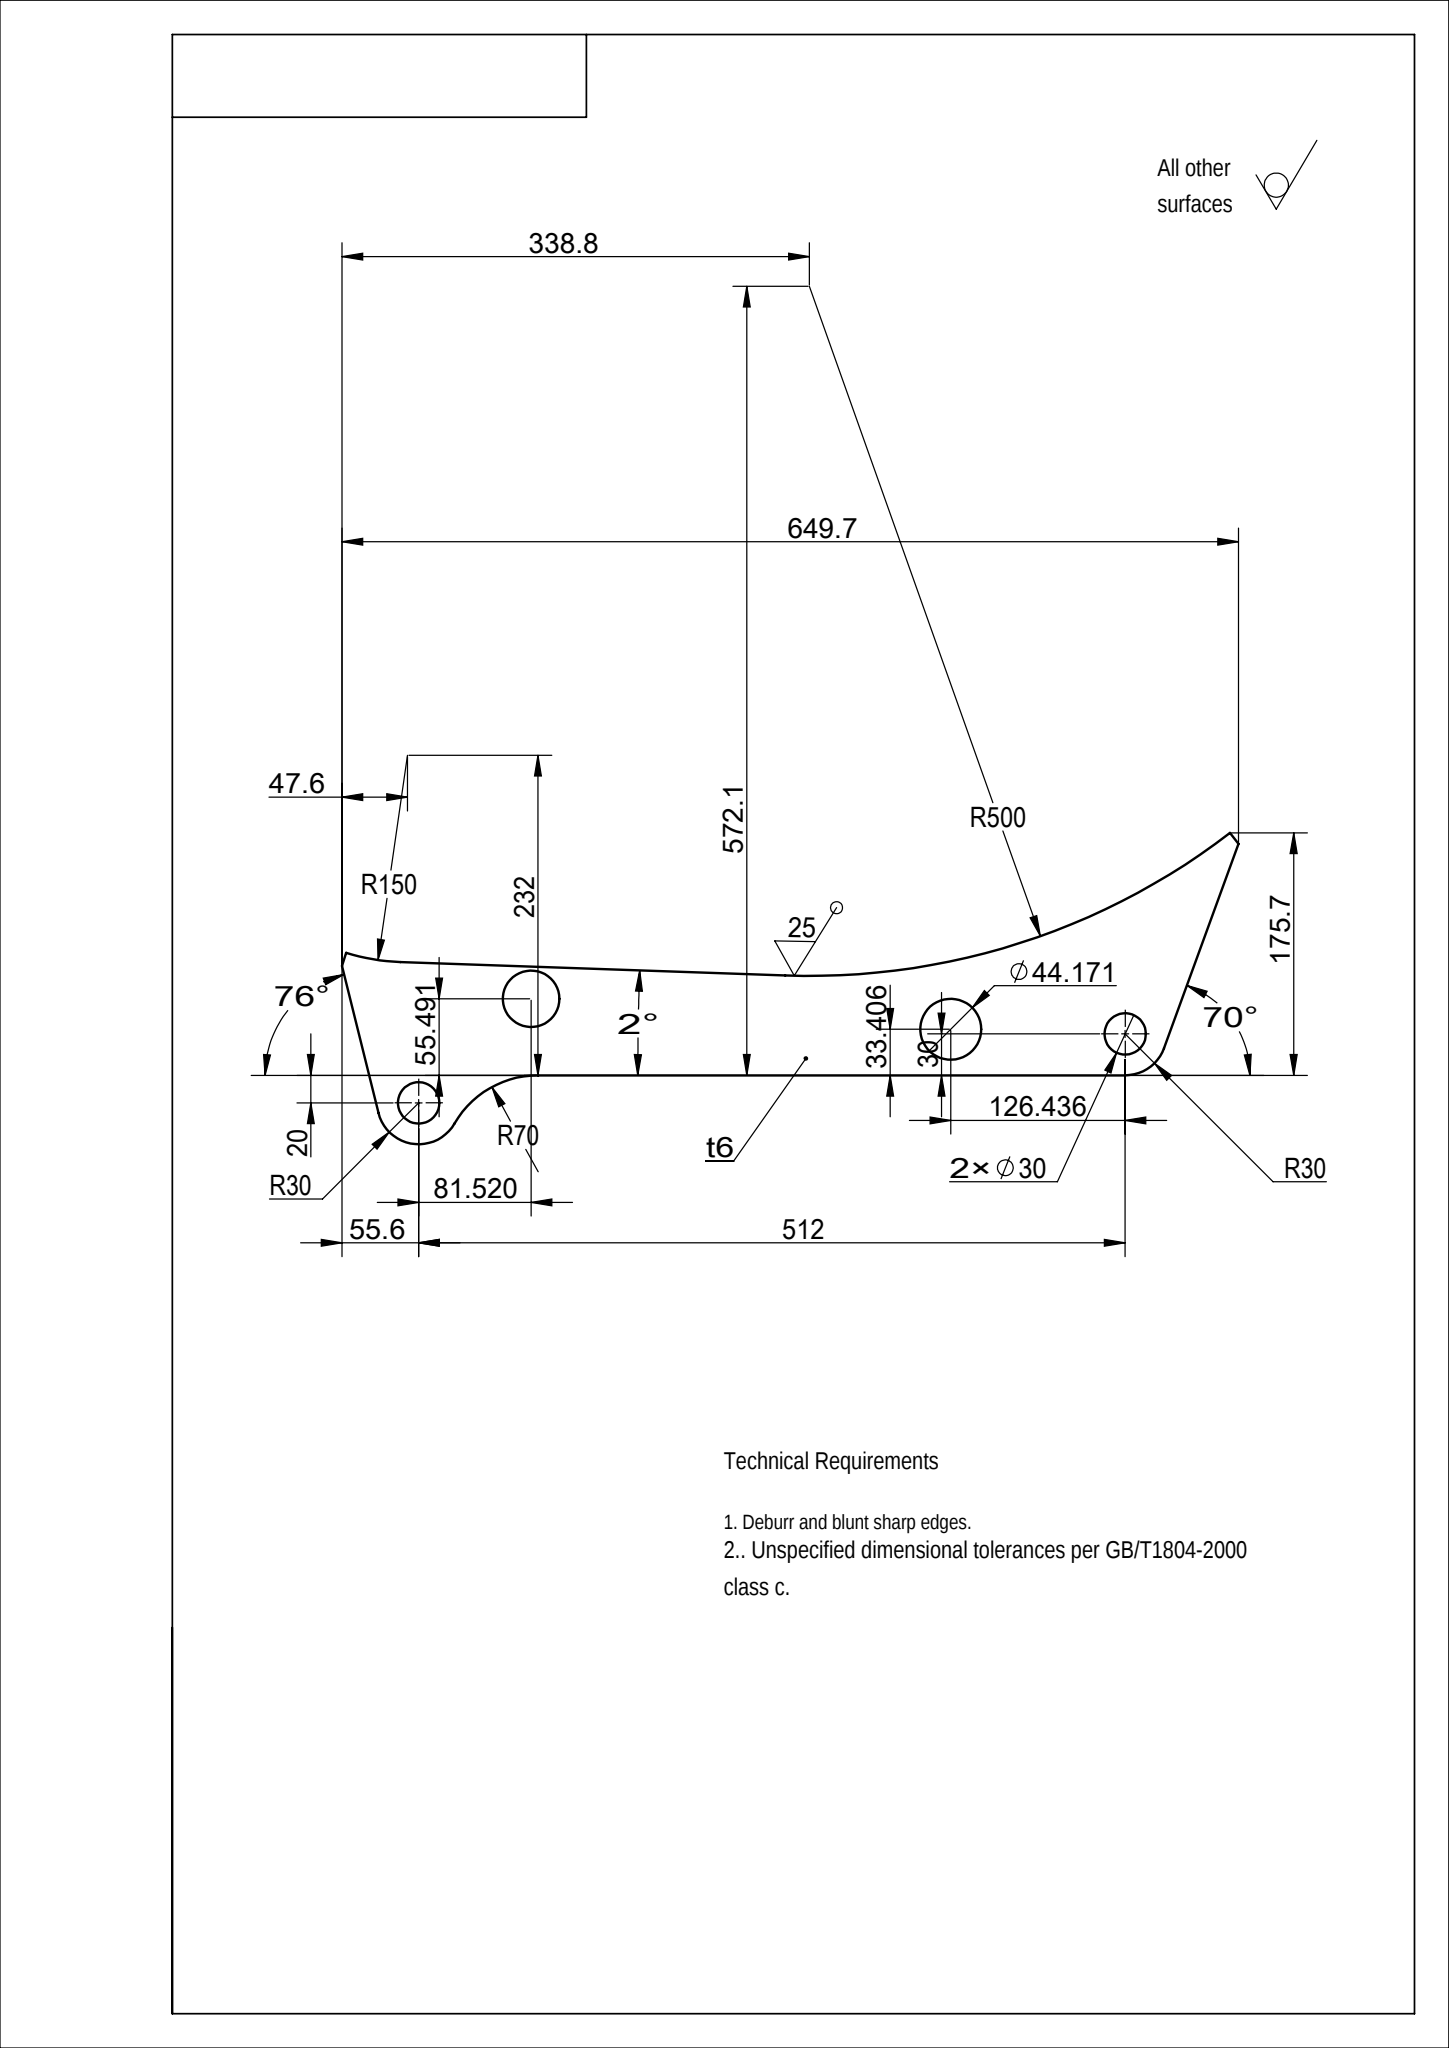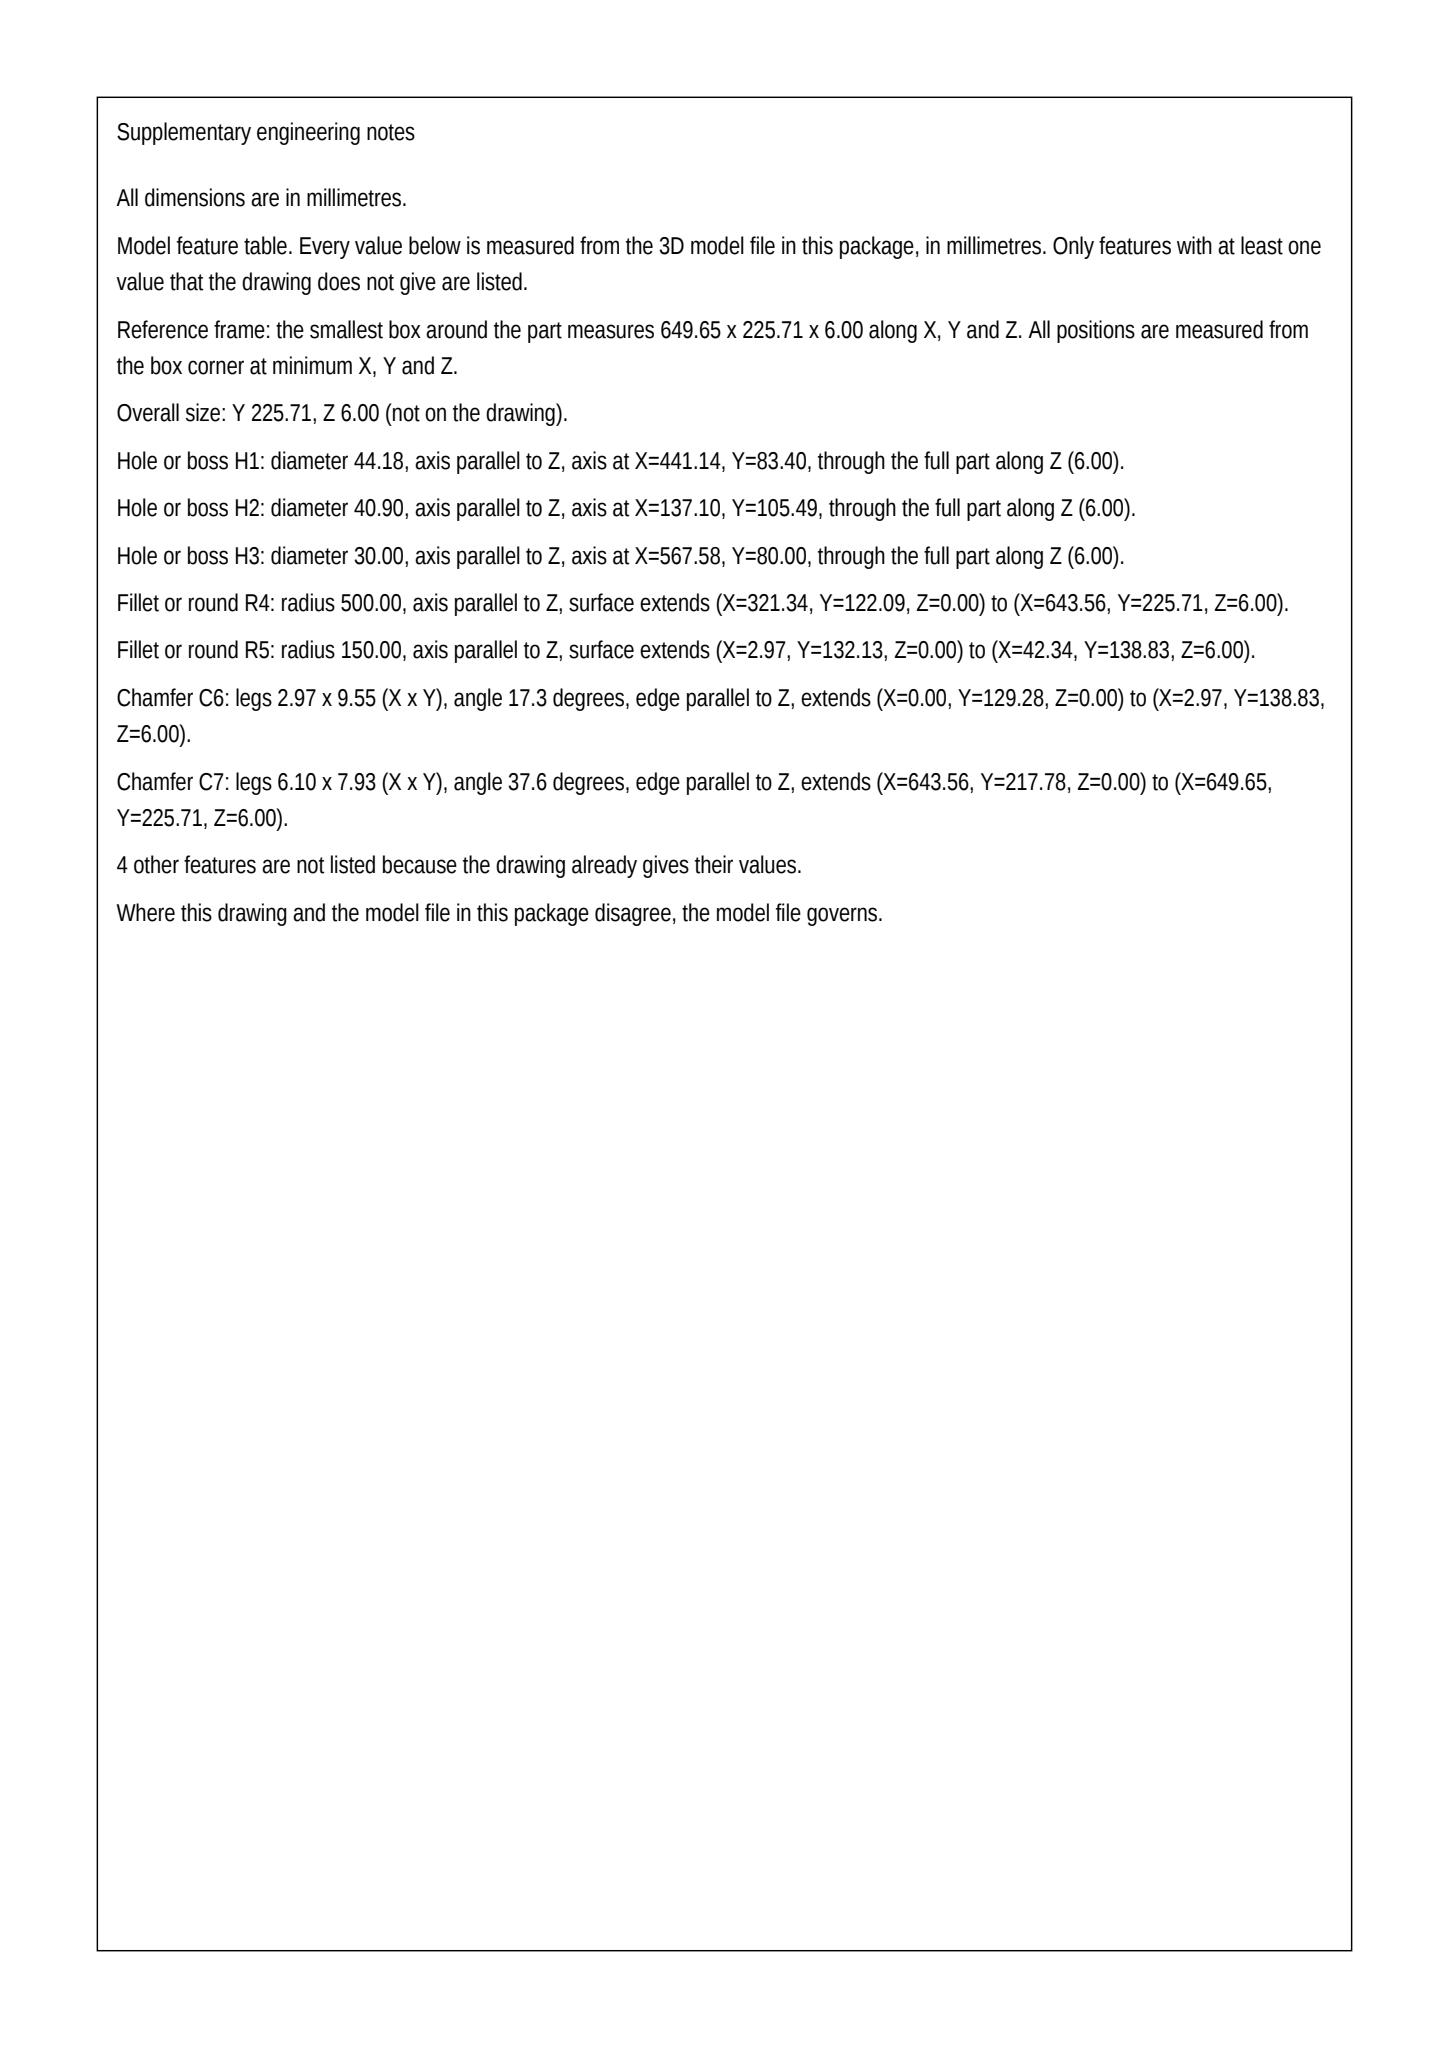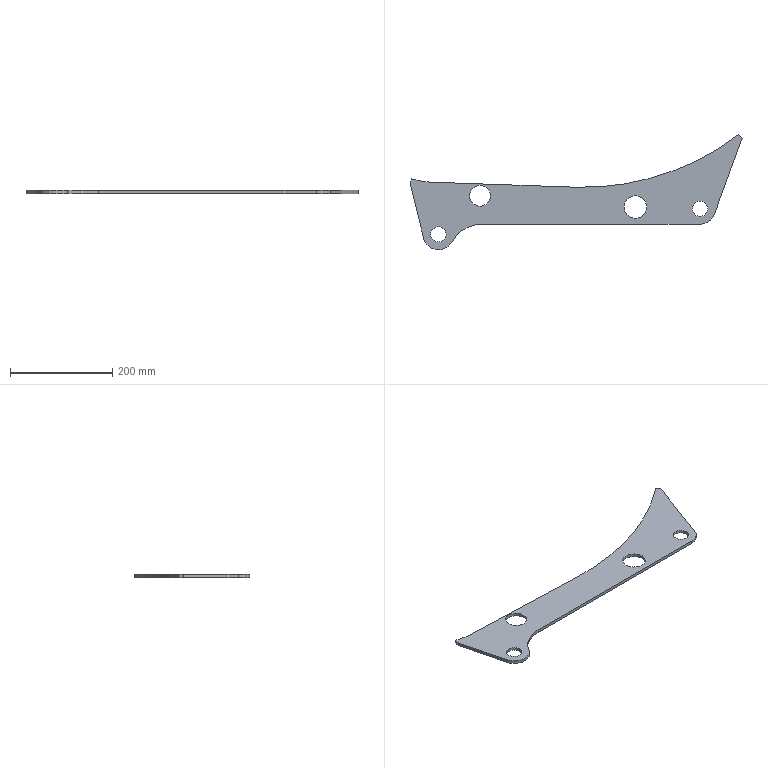Part | SolidWorks | mm | 1 solid | 21 faces | box 649.65 x 225.71 x 6 mm | volume 314367 mm3 | cylinder 13 | plane 8 | commonest cylinder face diameters 30 x4 44.171 x2 40.91 x2 60 x2 140 x1 1000 x1 300 x1
build123d program:
from build123d import *

# Parameters (mm, degrees)
BOSS_EXTRUDE1_START = 250
SKETCH1_R           = 15
BOSS_EXTRUDE1_DEPTH = 6
SKETCH3_R           = 22.086
SKETCH3_R_2         = 20.455
CUT_EXTRUDE2_DEPTH  = 80


with BuildPart() as part:
    # Sketch1 → Boss-Extrude1 (new body)
    with BuildSketch(Plane.XY.offset(BOSS_EXTRUDE1_START)):
        with BuildLine():
            Line((105.394, -627.925), (102.421, -637.473))
            Line((102.421, -637.473), (107.706, -658.746))
            Line((107.706, -658.746), (128.885, -743.987))
            ThreePointArc((128.885, -743.987), (153.813, -766.46), (183.981, -751.753))
            ThreePointArc((183.981, -751.753), (209.603, -726.132), (244.603, -716.753))
            Line((244.603, -716.753), (670, -716.753))
            ThreePointArc((670, -716.753), (687.207, -711.328), (698.191, -697.014))
            Line((698.191, -697.014), (752.073, -548.975))
            Line((752.073, -548.975), (745.977, -541.048))
            ThreePointArc((745.977, -541.048), (593.875, -620.791), (423.761, -644.363))
            Line((423.761, -644.363), (144.765, -634.62))
            ThreePointArc((144.765, -634.62), (124.856, -632.589), (105.394, -627.925))
        make_face()
        with Locations((670, -686.753)):
            Circle(SKETCH1_R, mode=Mode.SUBTRACT)
        with Locations((158, -736.753)):
            Circle(SKETCH1_R, mode=Mode.SUBTRACT)
    extrude(amount=BOSS_EXTRUDE1_DEPTH)

    # Sketch3 → Cut-Extrude2 (cut)
    with BuildSketch(Plane(origin=(0, 0, 250), x_dir=(-1, 0, 0), z_dir=(0, 0, -1))):
        with Locations((-543.564, -683.348)):
            Circle(SKETCH3_R)
        with Locations((-239.52, -661.262)):
            Circle(SKETCH3_R_2)
    extrude(amount=-CUT_EXTRUDE2_DEPTH, mode=Mode.SUBTRACT)


solid = part.part
STEP:
#1=CARTESIAN_POINT('',(521.478,-683.348,256.));
#2=VERTEX_POINT('',#1);
#3=CARTESIAN_POINT('',(565.649,-683.348,256.));
#4=VERTEX_POINT('',#3);
#5=CARTESIAN_POINT('',(543.564,-683.348,256.));
#6=DIRECTION('',(0.,0.,1.));
#7=DIRECTION('',(1.,0.,0.));
#8=AXIS2_PLACEMENT_3D('',#5,#6,#7);
#9=CIRCLE('',#8,22.086);
#10=EDGE_CURVE('',#2,#4,#9,.T.);
#11=ORIENTED_EDGE('',*,*,#10,.T.);
#12=CARTESIAN_POINT('',(565.649,-683.348,250.));
#13=VERTEX_POINT('',#12);
#14=CARTESIAN_POINT('',(565.649,-683.348,330.));
#15=DIRECTION('',(0.,0.,-1.));
#16=VECTOR('',#15,1000.);
#17=LINE('',#14,#16);
#18=EDGE_CURVE('',#4,#13,#17,.T.);
#19=ORIENTED_EDGE('',*,*,#18,.T.);
#20=CARTESIAN_POINT('',(521.478,-683.348,250.));
#21=VERTEX_POINT('',#20);
#22=CARTESIAN_POINT('',(543.564,-683.348,250.));
#23=DIRECTION('',(0.,0.,-1.));
#24=DIRECTION('',(-1.,0.,0.));
#25=AXIS2_PLACEMENT_3D('',#22,#23,#24);
#26=CIRCLE('',#25,22.086);
#27=EDGE_CURVE('',#13,#21,#26,.T.);
#28=ORIENTED_EDGE('',*,*,#27,.T.);
#29=CARTESIAN_POINT('',(521.478,-683.348,330.));
#30=DIRECTION('',(0.,0.,-1.));
#31=VECTOR('',#30,1000.);
#32=LINE('',#29,#31);
#33=EDGE_CURVE('',#2,#21,#32,.T.);
#34=ORIENTED_EDGE('',*,*,#33,.F.);
#35=EDGE_LOOP('',(#11,#19,#28,#34));
#36=FACE_OUTER_BOUND('',#35,.T.);
#37=CARTESIAN_POINT('',(543.564,-683.348,330.));
#38=DIRECTION('',(0.,0.,-1.));
#39=DIRECTION('',(-1.,0.,0.));
#40=AXIS2_PLACEMENT_3D('',#37,#38,#39);
#41=CYLINDRICAL_SURFACE('',#40,22.086);
#42=ADVANCED_FACE('',(#36),#41,.F.);
#43=CARTESIAN_POINT('',(219.065,-661.262,256.));
#44=VERTEX_POINT('',#43);
#45=CARTESIAN_POINT('',(259.975,-661.262,256.));
#46=VERTEX_POINT('',#45);
#47=CARTESIAN_POINT('',(239.52,-661.262,256.));
#48=DIRECTION('',(0.,0.,1.));
#49=DIRECTION('',(1.,0.,0.));
#50=AXIS2_PLACEMENT_3D('',#47,#48,#49);
#51=CIRCLE('',#50,20.455);
#52=EDGE_CURVE('',#44,#46,#51,.T.);
#53=ORIENTED_EDGE('',*,*,#52,.T.);
#54=CARTESIAN_POINT('',(259.975,-661.262,250.));
#55=VERTEX_POINT('',#54);
#56=CARTESIAN_POINT('',(259.975,-661.262,330.));
#57=DIRECTION('',(0.,0.,-1.));
#58=VECTOR('',#57,1000.);
#59=LINE('',#56,#58);
#60=EDGE_CURVE('',#46,#55,#59,.T.);
#61=ORIENTED_EDGE('',*,*,#60,.T.);
#62=CARTESIAN_POINT('',(219.065,-661.262,250.));
#63=VERTEX_POINT('',#62);
#64=CARTESIAN_POINT('',(239.52,-661.262,250.));
#65=DIRECTION('',(0.,0.,-1.));
#66=DIRECTION('',(-1.,0.,0.));
#67=AXIS2_PLACEMENT_3D('',#64,#65,#66);
#68=CIRCLE('',#67,20.455);
#69=EDGE_CURVE('',#55,#63,#68,.T.);
#70=ORIENTED_EDGE('',*,*,#69,.T.);
#71=CARTESIAN_POINT('',(219.065,-661.262,330.));
#72=DIRECTION('',(0.,0.,-1.));
#73=VECTOR('',#72,1000.);
#74=LINE('',#71,#73);
#75=EDGE_CURVE('',#44,#63,#74,.T.);
#76=ORIENTED_EDGE('',*,*,#75,.F.);
#77=EDGE_LOOP('',(#53,#61,#70,#76));
#78=FACE_OUTER_BOUND('',#77,.T.);
#79=CARTESIAN_POINT('',(239.52,-661.262,330.));
#80=DIRECTION('',(0.,0.,-1.));
#81=DIRECTION('',(-1.,0.,0.));
#82=AXIS2_PLACEMENT_3D('',#79,#80,#81);
#83=CYLINDRICAL_SURFACE('',#82,20.455);
#84=ADVANCED_FACE('',(#78),#83,.F.);
#85=CARTESIAN_POINT('',(143.,-736.753,256.));
#86=VERTEX_POINT('',#85);
#87=CARTESIAN_POINT('',(173.,-736.753,256.));
#88=VERTEX_POINT('',#87);
#89=CARTESIAN_POINT('',(158.,-736.753,256.));
#90=DIRECTION('',(0.,0.,1.));
#91=DIRECTION('',(1.,0.,0.));
#92=AXIS2_PLACEMENT_3D('',#89,#90,#91);
#93=CIRCLE('',#92,15.);
#94=EDGE_CURVE('',#86,#88,#93,.T.);
#95=ORIENTED_EDGE('',*,*,#94,.T.);
#96=CARTESIAN_POINT('',(173.,-736.753,250.));
#97=VERTEX_POINT('',#96);
#98=CARTESIAN_POINT('',(173.,-736.753,256.));
#99=DIRECTION('',(0.,0.,-1.));
#100=VECTOR('',#99,1000.);
#101=LINE('',#98,#100);
#102=EDGE_CURVE('',#88,#97,#101,.T.);
#103=ORIENTED_EDGE('',*,*,#102,.T.);
#104=CARTESIAN_POINT('',(143.,-736.753,250.));
#105=VERTEX_POINT('',#104);
#106=CARTESIAN_POINT('',(158.,-736.753,250.));
#107=DIRECTION('',(0.,0.,1.));
#108=DIRECTION('',(1.,0.,0.));
#109=AXIS2_PLACEMENT_3D('',#106,#107,#108);
#110=CIRCLE('',#109,15.);
#111=EDGE_CURVE('',#105,#97,#110,.T.);
#112=ORIENTED_EDGE('',*,*,#111,.F.);
#113=CARTESIAN_POINT('',(143.,-736.753,256.));
#114=DIRECTION('',(0.,0.,-1.));
#115=VECTOR('',#114,1000.);
#116=LINE('',#113,#115);
#117=EDGE_CURVE('',#86,#105,#116,.T.);
#118=ORIENTED_EDGE('',*,*,#117,.F.);
#119=EDGE_LOOP('',(#95,#103,#112,#118));
#120=FACE_OUTER_BOUND('',#119,.T.);
#121=CARTESIAN_POINT('',(158.,-736.753,256.));
#122=DIRECTION('',(0.,0.,-1.));
#123=DIRECTION('',(-1.,0.,0.));
#124=AXIS2_PLACEMENT_3D('',#121,#122,#123);
#125=CYLINDRICAL_SURFACE('',#124,15.);
#126=ADVANCED_FACE('',(#120),#125,.F.);
#127=CARTESIAN_POINT('',(655.,-686.753,256.));
#128=VERTEX_POINT('',#127);
#129=CARTESIAN_POINT('',(685.,-686.753,256.));
#130=VERTEX_POINT('',#129);
#131=CARTESIAN_POINT('',(670.,-686.753,256.));
#132=DIRECTION('',(0.,0.,1.));
#133=DIRECTION('',(1.,0.,0.));
#134=AXIS2_PLACEMENT_3D('',#131,#132,#133);
#135=CIRCLE('',#134,15.);
#136=EDGE_CURVE('',#128,#130,#135,.T.);
#137=ORIENTED_EDGE('',*,*,#136,.T.);
#138=CARTESIAN_POINT('',(685.,-686.753,250.));
#139=VERTEX_POINT('',#138);
#140=CARTESIAN_POINT('',(685.,-686.753,256.));
#141=DIRECTION('',(0.,0.,-1.));
#142=VECTOR('',#141,1000.);
#143=LINE('',#140,#142);
#144=EDGE_CURVE('',#130,#139,#143,.T.);
#145=ORIENTED_EDGE('',*,*,#144,.T.);
#146=CARTESIAN_POINT('',(655.,-686.753,250.));
#147=VERTEX_POINT('',#146);
#148=CARTESIAN_POINT('',(670.,-686.753,250.));
#149=DIRECTION('',(0.,0.,1.));
#150=DIRECTION('',(1.,0.,0.));
#151=AXIS2_PLACEMENT_3D('',#148,#149,#150);
#152=CIRCLE('',#151,15.);
#153=EDGE_CURVE('',#147,#139,#152,.T.);
#154=ORIENTED_EDGE('',*,*,#153,.F.);
#155=CARTESIAN_POINT('',(655.,-686.753,256.));
#156=DIRECTION('',(0.,0.,-1.));
#157=VECTOR('',#156,1000.);
#158=LINE('',#155,#157);
#159=EDGE_CURVE('',#128,#147,#158,.T.);
#160=ORIENTED_EDGE('',*,*,#159,.F.);
#161=EDGE_LOOP('',(#137,#145,#154,#160));
#162=FACE_OUTER_BOUND('',#161,.T.);
#163=CARTESIAN_POINT('',(670.,-686.753,256.));
#164=DIRECTION('',(0.,0.,-1.));
#165=DIRECTION('',(-1.,0.,0.));
#166=AXIS2_PLACEMENT_3D('',#163,#164,#165);
#167=CYLINDRICAL_SURFACE('',#166,15.);
#168=ADVANCED_FACE('',(#162),#167,.F.);
#169=ORIENTED_EDGE('',*,*,#10,.F.);
#170=CARTESIAN_POINT('',(543.564,-683.348,256.));
#171=DIRECTION('',(0.,0.,1.));
#172=DIRECTION('',(1.,0.,0.));
#173=AXIS2_PLACEMENT_3D('',#170,#171,#172);
#174=CIRCLE('',#173,22.086);
#175=EDGE_CURVE('',#4,#2,#174,.T.);
#176=ORIENTED_EDGE('',*,*,#175,.F.);
#177=EDGE_LOOP('',(#169,#176));
#178=FACE_BOUND('',#177,.T.);
#179=ORIENTED_EDGE('',*,*,#52,.F.);
#180=CARTESIAN_POINT('',(239.52,-661.262,256.));
#181=DIRECTION('',(0.,0.,1.));
#182=DIRECTION('',(1.,0.,0.));
#183=AXIS2_PLACEMENT_3D('',#180,#181,#182);
#184=CIRCLE('',#183,20.455);
#185=EDGE_CURVE('',#46,#44,#184,.T.);
#186=ORIENTED_EDGE('',*,*,#185,.F.);
#187=EDGE_LOOP('',(#179,#186));
#188=FACE_BOUND('',#187,.T.);
#189=ORIENTED_EDGE('',*,*,#136,.F.);
#190=CARTESIAN_POINT('',(670.,-686.753,256.));
#191=DIRECTION('',(0.,0.,1.));
#192=DIRECTION('',(1.,0.,0.));
#193=AXIS2_PLACEMENT_3D('',#190,#191,#192);
#194=CIRCLE('',#193,15.);
#195=EDGE_CURVE('',#130,#128,#194,.T.);
#196=ORIENTED_EDGE('',*,*,#195,.F.);
#197=EDGE_LOOP('',(#189,#196));
#198=FACE_BOUND('',#197,.T.);
#199=CARTESIAN_POINT('',(102.421,-637.473,256.));
#200=VERTEX_POINT('',#199);
#201=CARTESIAN_POINT('',(128.885,-743.987,256.));
#202=VERTEX_POINT('',#201);
#203=CARTESIAN_POINT('',(102.421,-637.473,256.));
#204=DIRECTION('',(0.2411,-0.9705,0.));
#205=VECTOR('',#204,1000.);
#206=LINE('',#203,#205);
#207=EDGE_CURVE('',#200,#202,#206,.T.);
#208=ORIENTED_EDGE('',*,*,#207,.T.);
#209=CARTESIAN_POINT('',(183.981,-751.753,256.));
#210=VERTEX_POINT('',#209);
#211=CARTESIAN_POINT('',(158.,-736.753,256.));
#212=DIRECTION('',(0.,0.,1.));
#213=DIRECTION('',(1.,0.,0.));
#214=AXIS2_PLACEMENT_3D('',#211,#212,#213);
#215=CIRCLE('',#214,30.);
#216=EDGE_CURVE('',#202,#210,#215,.T.);
#217=ORIENTED_EDGE('',*,*,#216,.T.);
#218=CARTESIAN_POINT('',(244.603,-716.753,256.));
#219=VERTEX_POINT('',#218);
#220=CARTESIAN_POINT('',(244.603,-786.753,256.));
#221=DIRECTION('',(0.,0.,-1.));
#222=DIRECTION('',(-1.,0.,0.));
#223=AXIS2_PLACEMENT_3D('',#220,#221,#222);
#224=CIRCLE('',#223,70.);
#225=EDGE_CURVE('',#210,#219,#224,.T.);
#226=ORIENTED_EDGE('',*,*,#225,.T.);
#227=CARTESIAN_POINT('',(670.,-716.753,256.));
#228=VERTEX_POINT('',#227);
#229=CARTESIAN_POINT('',(244.603,-716.753,256.));
#230=DIRECTION('',(1.,0.,0.));
#231=VECTOR('',#230,1000.);
#232=LINE('',#229,#231);
#233=EDGE_CURVE('',#219,#228,#232,.T.);
#234=ORIENTED_EDGE('',*,*,#233,.T.);
#235=CARTESIAN_POINT('',(698.191,-697.014,256.));
#236=VERTEX_POINT('',#235);
#237=CARTESIAN_POINT('',(670.,-686.753,256.));
#238=DIRECTION('',(0.,0.,1.));
#239=DIRECTION('',(1.,0.,0.));
#240=AXIS2_PLACEMENT_3D('',#237,#238,#239);
#241=CIRCLE('',#240,30.);
#242=EDGE_CURVE('',#228,#236,#241,.T.);
#243=ORIENTED_EDGE('',*,*,#242,.T.);
#244=CARTESIAN_POINT('',(752.073,-548.975,256.));
#245=VERTEX_POINT('',#244);
#246=CARTESIAN_POINT('',(698.191,-697.014,256.));
#247=DIRECTION('',(0.342,0.9397,0.));
#248=VECTOR('',#247,1000.);
#249=LINE('',#246,#248);
#250=EDGE_CURVE('',#236,#245,#249,.T.);
#251=ORIENTED_EDGE('',*,*,#250,.T.);
#252=CARTESIAN_POINT('',(745.977,-541.048,256.));
#253=VERTEX_POINT('',#252);
#254=CARTESIAN_POINT('',(752.073,-548.975,256.));
#255=DIRECTION('',(-0.6095,0.7928,0.));
#256=VECTOR('',#255,1000.);
#257=LINE('',#254,#256);
#258=EDGE_CURVE('',#245,#253,#257,.T.);
#259=ORIENTED_EDGE('',*,*,#258,.T.);
#260=CARTESIAN_POINT('',(423.761,-644.363,256.));
#261=VERTEX_POINT('',#260);
#262=CARTESIAN_POINT('',(441.211,-144.667,256.));
#263=DIRECTION('',(0.,0.,-1.));
#264=DIRECTION('',(-1.,0.,0.));
#265=AXIS2_PLACEMENT_3D('',#262,#263,#264);
#266=CIRCLE('',#265,500.);
#267=EDGE_CURVE('',#253,#261,#266,.T.);
#268=ORIENTED_EDGE('',*,*,#267,.T.);
#269=CARTESIAN_POINT('',(144.765,-634.62,256.));
#270=VERTEX_POINT('',#269);
#271=CARTESIAN_POINT('',(423.761,-644.363,256.));
#272=DIRECTION('',(-0.9994,0.0349,0.));
#273=VECTOR('',#272,1000.);
#274=LINE('',#271,#273);
#275=EDGE_CURVE('',#261,#270,#274,.T.);
#276=ORIENTED_EDGE('',*,*,#275,.T.);
#277=CARTESIAN_POINT('',(105.394,-627.925,256.));
#278=VERTEX_POINT('',#277);
#279=CARTESIAN_POINT('',(150.,-484.711,256.));
#280=DIRECTION('',(0.,0.,-1.));
#281=DIRECTION('',(-1.,0.,0.));
#282=AXIS2_PLACEMENT_3D('',#279,#280,#281);
#283=CIRCLE('',#282,150.);
#284=EDGE_CURVE('',#270,#278,#283,.T.);
#285=ORIENTED_EDGE('',*,*,#284,.T.);
#286=CARTESIAN_POINT('',(105.394,-627.925,256.));
#287=DIRECTION('',(-0.2974,-0.9548,0.));
#288=VECTOR('',#287,1000.);
#289=LINE('',#286,#288);
#290=EDGE_CURVE('',#278,#200,#289,.T.);
#291=ORIENTED_EDGE('',*,*,#290,.T.);
#292=EDGE_LOOP('',(#208,#217,#226,#234,#243,#251,#259,#268,#276,#285,#291));
#293=FACE_OUTER_BOUND('',#292,.T.);
#294=ORIENTED_EDGE('',*,*,#94,.F.);
#295=CARTESIAN_POINT('',(158.,-736.753,256.));
#296=DIRECTION('',(0.,0.,1.));
#297=DIRECTION('',(1.,0.,0.));
#298=AXIS2_PLACEMENT_3D('',#295,#296,#297);
#299=CIRCLE('',#298,15.);
#300=EDGE_CURVE('',#88,#86,#299,.T.);
#301=ORIENTED_EDGE('',*,*,#300,.F.);
#302=EDGE_LOOP('',(#294,#301));
#303=FACE_BOUND('',#302,.T.);
#304=CARTESIAN_POINT('',(158.,-736.753,256.));
#305=DIRECTION('',(0.,0.,1.));
#306=DIRECTION('',(1.,0.,0.));
#307=AXIS2_PLACEMENT_3D('',#304,#305,#306);
#308=PLANE('',#307);
#309=ADVANCED_FACE('',(#178,#188,#198,#293,#303),#308,.T.);
#310=CARTESIAN_POINT('',(543.564,-683.348,250.));
#311=DIRECTION('',(0.,0.,-1.));
#312=DIRECTION('',(-1.,0.,0.));
#313=AXIS2_PLACEMENT_3D('',#310,#311,#312);
#314=CIRCLE('',#313,22.086);
#315=EDGE_CURVE('',#21,#13,#314,.T.);
#316=ORIENTED_EDGE('',*,*,#315,.F.);
#317=ORIENTED_EDGE('',*,*,#27,.F.);
#318=EDGE_LOOP('',(#316,#317));
#319=FACE_BOUND('',#318,.T.);
#320=CARTESIAN_POINT('',(239.52,-661.262,250.));
#321=DIRECTION('',(0.,0.,-1.));
#322=DIRECTION('',(-1.,0.,0.));
#323=AXIS2_PLACEMENT_3D('',#320,#321,#322);
#324=CIRCLE('',#323,20.455);
#325=EDGE_CURVE('',#63,#55,#324,.T.);
#326=ORIENTED_EDGE('',*,*,#325,.F.);
#327=ORIENTED_EDGE('',*,*,#69,.F.);
#328=EDGE_LOOP('',(#326,#327));
#329=FACE_BOUND('',#328,.T.);
#330=CARTESIAN_POINT('',(102.421,-637.473,250.));
#331=VERTEX_POINT('',#330);
#332=CARTESIAN_POINT('',(128.885,-743.987,250.));
#333=VERTEX_POINT('',#332);
#334=CARTESIAN_POINT('',(107.706,-658.746,250.));
#335=DIRECTION('',(0.2411,-0.9705,0.));
#336=VECTOR('',#335,1000.);
#337=LINE('',#334,#336);
#338=EDGE_CURVE('',#331,#333,#337,.T.);
#339=ORIENTED_EDGE('',*,*,#338,.F.);
#340=CARTESIAN_POINT('',(105.394,-627.925,250.));
#341=VERTEX_POINT('',#340);
#342=CARTESIAN_POINT('',(105.394,-627.925,250.));
#343=DIRECTION('',(-0.2974,-0.9548,0.));
#344=VECTOR('',#343,1000.);
#345=LINE('',#342,#344);
#346=EDGE_CURVE('',#341,#331,#345,.T.);
#347=ORIENTED_EDGE('',*,*,#346,.F.);
#348=CARTESIAN_POINT('',(144.765,-634.62,250.));
#349=VERTEX_POINT('',#348);
#350=CARTESIAN_POINT('',(150.,-484.711,250.));
#351=DIRECTION('',(0.,0.,-1.));
#352=DIRECTION('',(-1.,0.,0.));
#353=AXIS2_PLACEMENT_3D('',#350,#351,#352);
#354=CIRCLE('',#353,150.);
#355=EDGE_CURVE('',#349,#341,#354,.T.);
#356=ORIENTED_EDGE('',*,*,#355,.F.);
#357=CARTESIAN_POINT('',(423.761,-644.363,250.));
#358=VERTEX_POINT('',#357);
#359=CARTESIAN_POINT('',(423.761,-644.363,250.));
#360=DIRECTION('',(-0.9994,0.0349,0.));
#361=VECTOR('',#360,1000.);
#362=LINE('',#359,#361);
#363=EDGE_CURVE('',#358,#349,#362,.T.);
#364=ORIENTED_EDGE('',*,*,#363,.F.);
#365=CARTESIAN_POINT('',(745.977,-541.048,250.));
#366=VERTEX_POINT('',#365);
#367=CARTESIAN_POINT('',(441.211,-144.667,250.));
#368=DIRECTION('',(0.,0.,-1.));
#369=DIRECTION('',(-1.,0.,0.));
#370=AXIS2_PLACEMENT_3D('',#367,#368,#369);
#371=CIRCLE('',#370,500.);
#372=EDGE_CURVE('',#366,#358,#371,.T.);
#373=ORIENTED_EDGE('',*,*,#372,.F.);
#374=CARTESIAN_POINT('',(752.073,-548.975,250.));
#375=VERTEX_POINT('',#374);
#376=CARTESIAN_POINT('',(752.073,-548.975,250.));
#377=DIRECTION('',(-0.6095,0.7928,0.));
#378=VECTOR('',#377,1000.);
#379=LINE('',#376,#378);
#380=EDGE_CURVE('',#375,#366,#379,.T.);
#381=ORIENTED_EDGE('',*,*,#380,.F.);
#382=CARTESIAN_POINT('',(698.191,-697.014,250.));
#383=VERTEX_POINT('',#382);
#384=CARTESIAN_POINT('',(698.191,-697.014,250.));
#385=DIRECTION('',(0.342,0.9397,0.));
#386=VECTOR('',#385,1000.);
#387=LINE('',#384,#386);
#388=EDGE_CURVE('',#383,#375,#387,.T.);
#389=ORIENTED_EDGE('',*,*,#388,.F.);
#390=CARTESIAN_POINT('',(670.,-716.753,250.));
#391=VERTEX_POINT('',#390);
#392=CARTESIAN_POINT('',(670.,-686.753,250.));
#393=DIRECTION('',(0.,0.,1.));
#394=DIRECTION('',(1.,0.,0.));
#395=AXIS2_PLACEMENT_3D('',#392,#393,#394);
#396=CIRCLE('',#395,30.);
#397=EDGE_CURVE('',#391,#383,#396,.T.);
#398=ORIENTED_EDGE('',*,*,#397,.F.);
#399=CARTESIAN_POINT('',(244.603,-716.753,250.));
#400=VERTEX_POINT('',#399);
#401=CARTESIAN_POINT('',(244.603,-716.753,250.));
#402=DIRECTION('',(1.,0.,0.));
#403=VECTOR('',#402,1000.);
#404=LINE('',#401,#403);
#405=EDGE_CURVE('',#400,#391,#404,.T.);
#406=ORIENTED_EDGE('',*,*,#405,.F.);
#407=CARTESIAN_POINT('',(183.981,-751.753,250.));
#408=VERTEX_POINT('',#407);
#409=CARTESIAN_POINT('',(244.603,-786.753,250.));
#410=DIRECTION('',(0.,0.,-1.));
#411=DIRECTION('',(-1.,0.,0.));
#412=AXIS2_PLACEMENT_3D('',#409,#410,#411);
#413=CIRCLE('',#412,70.);
#414=EDGE_CURVE('',#408,#400,#413,.T.);
#415=ORIENTED_EDGE('',*,*,#414,.F.);
#416=CARTESIAN_POINT('',(158.,-736.753,250.));
#417=DIRECTION('',(0.,0.,1.));
#418=DIRECTION('',(1.,0.,0.));
#419=AXIS2_PLACEMENT_3D('',#416,#417,#418);
#420=CIRCLE('',#419,30.);
#421=EDGE_CURVE('',#333,#408,#420,.T.);
#422=ORIENTED_EDGE('',*,*,#421,.F.);
#423=EDGE_LOOP('',(#339,#347,#356,#364,#373,#381,#389,#398,#406,#415,#422));
#424=FACE_OUTER_BOUND('',#423,.T.);
#425=ORIENTED_EDGE('',*,*,#153,.T.);
#426=CARTESIAN_POINT('',(670.,-686.753,250.));
#427=DIRECTION('',(0.,0.,1.));
#428=DIRECTION('',(1.,0.,0.));
#429=AXIS2_PLACEMENT_3D('',#426,#427,#428);
#430=CIRCLE('',#429,15.);
#431=EDGE_CURVE('',#139,#147,#430,.T.);
#432=ORIENTED_EDGE('',*,*,#431,.T.);
#433=EDGE_LOOP('',(#425,#432));
#434=FACE_BOUND('',#433,.T.);
#435=ORIENTED_EDGE('',*,*,#111,.T.);
#436=CARTESIAN_POINT('',(158.,-736.753,250.));
#437=DIRECTION('',(0.,0.,1.));
#438=DIRECTION('',(1.,0.,0.));
#439=AXIS2_PLACEMENT_3D('',#436,#437,#438);
#440=CIRCLE('',#439,15.);
#441=EDGE_CURVE('',#97,#105,#440,.T.);
#442=ORIENTED_EDGE('',*,*,#441,.T.);
#443=EDGE_LOOP('',(#435,#442));
#444=FACE_BOUND('',#443,.T.);
#445=CARTESIAN_POINT('',(158.,-736.753,250.));
#446=DIRECTION('',(0.,0.,1.));
#447=DIRECTION('',(1.,0.,0.));
#448=AXIS2_PLACEMENT_3D('',#445,#446,#447);
#449=PLANE('',#448);
#450=ADVANCED_FACE('',(#319,#329,#424,#434,#444),#449,.F.);
#451=ORIENTED_EDGE('',*,*,#338,.T.);
#452=CARTESIAN_POINT('',(128.885,-743.987,256.));
#453=DIRECTION('',(0.,0.,-1.));
#454=VECTOR('',#453,1000.);
#455=LINE('',#452,#454);
#456=EDGE_CURVE('',#202,#333,#455,.T.);
#457=ORIENTED_EDGE('',*,*,#456,.F.);
#458=ORIENTED_EDGE('',*,*,#207,.F.);
#459=CARTESIAN_POINT('',(102.421,-637.473,256.));
#460=DIRECTION('',(0.,0.,-1.));
#461=VECTOR('',#460,1000.);
#462=LINE('',#459,#461);
#463=EDGE_CURVE('',#200,#331,#462,.T.);
#464=ORIENTED_EDGE('',*,*,#463,.T.);
#465=EDGE_LOOP('',(#451,#457,#458,#464));
#466=FACE_OUTER_BOUND('',#465,.T.);
#467=CARTESIAN_POINT('',(107.706,-658.746,256.));
#468=DIRECTION('',(0.9705,0.2411,0.));
#469=DIRECTION('',(-0.2411,0.9705,0.));
#470=AXIS2_PLACEMENT_3D('',#467,#468,#469);
#471=PLANE('',#470);
#472=ADVANCED_FACE('',(#466),#471,.F.);
#473=ORIENTED_EDGE('',*,*,#421,.T.);
#474=CARTESIAN_POINT('',(183.981,-751.753,256.));
#475=DIRECTION('',(0.,0.,-1.));
#476=VECTOR('',#475,1000.);
#477=LINE('',#474,#476);
#478=EDGE_CURVE('',#210,#408,#477,.T.);
#479=ORIENTED_EDGE('',*,*,#478,.F.);
#480=ORIENTED_EDGE('',*,*,#216,.F.);
#481=ORIENTED_EDGE('',*,*,#456,.T.);
#482=EDGE_LOOP('',(#473,#479,#480,#481));
#483=FACE_OUTER_BOUND('',#482,.T.);
#484=CARTESIAN_POINT('',(158.,-736.753,256.));
#485=DIRECTION('',(0.,0.,-1.));
#486=DIRECTION('',(-1.,0.,0.));
#487=AXIS2_PLACEMENT_3D('',#484,#485,#486);
#488=CYLINDRICAL_SURFACE('',#487,30.);
#489=ADVANCED_FACE('',(#483),#488,.T.);
#490=ORIENTED_EDGE('',*,*,#414,.T.);
#491=CARTESIAN_POINT('',(244.603,-716.753,256.));
#492=DIRECTION('',(0.,0.,-1.));
#493=VECTOR('',#492,1000.);
#494=LINE('',#491,#493);
#495=EDGE_CURVE('',#219,#400,#494,.T.);
#496=ORIENTED_EDGE('',*,*,#495,.F.);
#497=ORIENTED_EDGE('',*,*,#225,.F.);
#498=ORIENTED_EDGE('',*,*,#478,.T.);
#499=EDGE_LOOP('',(#490,#496,#497,#498));
#500=FACE_OUTER_BOUND('',#499,.T.);
#501=CARTESIAN_POINT('',(244.603,-786.753,256.));
#502=DIRECTION('',(0.,0.,-1.));
#503=DIRECTION('',(-1.,0.,0.));
#504=AXIS2_PLACEMENT_3D('',#501,#502,#503);
#505=CYLINDRICAL_SURFACE('',#504,70.);
#506=ADVANCED_FACE('',(#500),#505,.F.);
#507=ORIENTED_EDGE('',*,*,#405,.T.);
#508=CARTESIAN_POINT('',(670.,-716.753,256.));
#509=DIRECTION('',(0.,0.,-1.));
#510=VECTOR('',#509,1000.);
#511=LINE('',#508,#510);
#512=EDGE_CURVE('',#228,#391,#511,.T.);
#513=ORIENTED_EDGE('',*,*,#512,.F.);
#514=ORIENTED_EDGE('',*,*,#233,.F.);
#515=ORIENTED_EDGE('',*,*,#495,.T.);
#516=EDGE_LOOP('',(#507,#513,#514,#515));
#517=FACE_OUTER_BOUND('',#516,.T.);
#518=CARTESIAN_POINT('',(244.603,-716.753,256.));
#519=DIRECTION('',(-0.,1.,0.));
#520=DIRECTION('',(-1.,-0.,0.));
#521=AXIS2_PLACEMENT_3D('',#518,#519,#520);
#522=PLANE('',#521);
#523=ADVANCED_FACE('',(#517),#522,.F.);
#524=ORIENTED_EDGE('',*,*,#397,.T.);
#525=CARTESIAN_POINT('',(698.191,-697.014,256.));
#526=DIRECTION('',(0.,0.,-1.));
#527=VECTOR('',#526,1000.);
#528=LINE('',#525,#527);
#529=EDGE_CURVE('',#236,#383,#528,.T.);
#530=ORIENTED_EDGE('',*,*,#529,.F.);
#531=ORIENTED_EDGE('',*,*,#242,.F.);
#532=ORIENTED_EDGE('',*,*,#512,.T.);
#533=EDGE_LOOP('',(#524,#530,#531,#532));
#534=FACE_OUTER_BOUND('',#533,.T.);
#535=CARTESIAN_POINT('',(670.,-686.753,256.));
#536=DIRECTION('',(0.,0.,-1.));
#537=DIRECTION('',(-1.,0.,0.));
#538=AXIS2_PLACEMENT_3D('',#535,#536,#537);
#539=CYLINDRICAL_SURFACE('',#538,30.);
#540=ADVANCED_FACE('',(#534),#539,.T.);
#541=ORIENTED_EDGE('',*,*,#388,.T.);
#542=CARTESIAN_POINT('',(752.073,-548.975,256.));
#543=DIRECTION('',(0.,0.,-1.));
#544=VECTOR('',#543,1000.);
#545=LINE('',#542,#544);
#546=EDGE_CURVE('',#245,#375,#545,.T.);
#547=ORIENTED_EDGE('',*,*,#546,.F.);
#548=ORIENTED_EDGE('',*,*,#250,.F.);
#549=ORIENTED_EDGE('',*,*,#529,.T.);
#550=EDGE_LOOP('',(#541,#547,#548,#549));
#551=FACE_OUTER_BOUND('',#550,.T.);
#552=CARTESIAN_POINT('',(698.191,-697.014,256.));
#553=DIRECTION('',(-0.9397,0.342,0.));
#554=DIRECTION('',(-0.342,-0.9397,0.));
#555=AXIS2_PLACEMENT_3D('',#552,#553,#554);
#556=PLANE('',#555);
#557=ADVANCED_FACE('',(#551),#556,.F.);
#558=ORIENTED_EDGE('',*,*,#380,.T.);
#559=CARTESIAN_POINT('',(745.977,-541.048,256.));
#560=DIRECTION('',(0.,0.,-1.));
#561=VECTOR('',#560,1000.);
#562=LINE('',#559,#561);
#563=EDGE_CURVE('',#253,#366,#562,.T.);
#564=ORIENTED_EDGE('',*,*,#563,.F.);
#565=ORIENTED_EDGE('',*,*,#258,.F.);
#566=ORIENTED_EDGE('',*,*,#546,.T.);
#567=EDGE_LOOP('',(#558,#564,#565,#566));
#568=FACE_OUTER_BOUND('',#567,.T.);
#569=CARTESIAN_POINT('',(752.073,-548.975,256.));
#570=DIRECTION('',(-0.7928,-0.6095,0.));
#571=DIRECTION('',(0.6095,-0.7928,0.));
#572=AXIS2_PLACEMENT_3D('',#569,#570,#571);
#573=PLANE('',#572);
#574=ADVANCED_FACE('',(#568),#573,.F.);
#575=ORIENTED_EDGE('',*,*,#372,.T.);
#576=CARTESIAN_POINT('',(423.761,-644.363,256.));
#577=DIRECTION('',(0.,0.,-1.));
#578=VECTOR('',#577,1000.);
#579=LINE('',#576,#578);
#580=EDGE_CURVE('',#261,#358,#579,.T.);
#581=ORIENTED_EDGE('',*,*,#580,.F.);
#582=ORIENTED_EDGE('',*,*,#267,.F.);
#583=ORIENTED_EDGE('',*,*,#563,.T.);
#584=EDGE_LOOP('',(#575,#581,#582,#583));
#585=FACE_OUTER_BOUND('',#584,.T.);
#586=CARTESIAN_POINT('',(441.211,-144.667,256.));
#587=DIRECTION('',(0.,0.,-1.));
#588=DIRECTION('',(-1.,0.,0.));
#589=AXIS2_PLACEMENT_3D('',#586,#587,#588);
#590=CYLINDRICAL_SURFACE('',#589,500.);
#591=ADVANCED_FACE('',(#585),#590,.F.);
#592=ORIENTED_EDGE('',*,*,#363,.T.);
#593=CARTESIAN_POINT('',(144.765,-634.62,256.));
#594=DIRECTION('',(0.,0.,-1.));
#595=VECTOR('',#594,1000.);
#596=LINE('',#593,#595);
#597=EDGE_CURVE('',#270,#349,#596,.T.);
#598=ORIENTED_EDGE('',*,*,#597,.F.);
#599=ORIENTED_EDGE('',*,*,#275,.F.);
#600=ORIENTED_EDGE('',*,*,#580,.T.);
#601=EDGE_LOOP('',(#592,#598,#599,#600));
#602=FACE_OUTER_BOUND('',#601,.T.);
#603=CARTESIAN_POINT('',(423.761,-644.363,256.));
#604=DIRECTION('',(-0.0349,-0.9994,0.));
#605=DIRECTION('',(0.9994,-0.0349,0.));
#606=AXIS2_PLACEMENT_3D('',#603,#604,#605);
#607=PLANE('',#606);
#608=ADVANCED_FACE('',(#602),#607,.F.);
#609=ORIENTED_EDGE('',*,*,#355,.T.);
#610=CARTESIAN_POINT('',(105.394,-627.925,256.));
#611=DIRECTION('',(0.,0.,-1.));
#612=VECTOR('',#611,1000.);
#613=LINE('',#610,#612);
#614=EDGE_CURVE('',#278,#341,#613,.T.);
#615=ORIENTED_EDGE('',*,*,#614,.F.);
#616=ORIENTED_EDGE('',*,*,#284,.F.);
#617=ORIENTED_EDGE('',*,*,#597,.T.);
#618=EDGE_LOOP('',(#609,#615,#616,#617));
#619=FACE_OUTER_BOUND('',#618,.T.);
#620=CARTESIAN_POINT('',(150.,-484.711,256.));
#621=DIRECTION('',(0.,0.,-1.));
#622=DIRECTION('',(-1.,0.,0.));
#623=AXIS2_PLACEMENT_3D('',#620,#621,#622);
#624=CYLINDRICAL_SURFACE('',#623,150.);
#625=ADVANCED_FACE('',(#619),#624,.F.);
#626=ORIENTED_EDGE('',*,*,#346,.T.);
#627=ORIENTED_EDGE('',*,*,#463,.F.);
#628=ORIENTED_EDGE('',*,*,#290,.F.);
#629=ORIENTED_EDGE('',*,*,#614,.T.);
#630=EDGE_LOOP('',(#626,#627,#628,#629));
#631=FACE_OUTER_BOUND('',#630,.T.);
#632=CARTESIAN_POINT('',(105.394,-627.925,256.));
#633=DIRECTION('',(0.9548,-0.2974,0.));
#634=DIRECTION('',(0.2974,0.9548,0.));
#635=AXIS2_PLACEMENT_3D('',#632,#633,#634);
#636=PLANE('',#635);
#637=ADVANCED_FACE('',(#631),#636,.F.);
#638=ORIENTED_EDGE('',*,*,#144,.F.);
#639=ORIENTED_EDGE('',*,*,#195,.T.);
#640=ORIENTED_EDGE('',*,*,#159,.T.);
#641=ORIENTED_EDGE('',*,*,#431,.F.);
#642=EDGE_LOOP('',(#638,#639,#640,#641));
#643=FACE_OUTER_BOUND('',#642,.T.);
#644=CARTESIAN_POINT('',(670.,-686.753,256.));
#645=DIRECTION('',(0.,0.,-1.));
#646=DIRECTION('',(-1.,0.,0.));
#647=AXIS2_PLACEMENT_3D('',#644,#645,#646);
#648=CYLINDRICAL_SURFACE('',#647,15.);
#649=ADVANCED_FACE('',(#643),#648,.F.);
#650=ORIENTED_EDGE('',*,*,#102,.F.);
#651=ORIENTED_EDGE('',*,*,#300,.T.);
#652=ORIENTED_EDGE('',*,*,#117,.T.);
#653=ORIENTED_EDGE('',*,*,#441,.F.);
#654=EDGE_LOOP('',(#650,#651,#652,#653));
#655=FACE_OUTER_BOUND('',#654,.T.);
#656=CARTESIAN_POINT('',(158.,-736.753,256.));
#657=DIRECTION('',(0.,0.,-1.));
#658=DIRECTION('',(-1.,0.,0.));
#659=AXIS2_PLACEMENT_3D('',#656,#657,#658);
#660=CYLINDRICAL_SURFACE('',#659,15.);
#661=ADVANCED_FACE('',(#655),#660,.F.);
#662=ORIENTED_EDGE('',*,*,#60,.F.);
#663=ORIENTED_EDGE('',*,*,#185,.T.);
#664=ORIENTED_EDGE('',*,*,#75,.T.);
#665=ORIENTED_EDGE('',*,*,#325,.T.);
#666=EDGE_LOOP('',(#662,#663,#664,#665));
#667=FACE_OUTER_BOUND('',#666,.T.);
#668=CARTESIAN_POINT('',(239.52,-661.262,330.));
#669=DIRECTION('',(0.,0.,-1.));
#670=DIRECTION('',(-1.,0.,0.));
#671=AXIS2_PLACEMENT_3D('',#668,#669,#670);
#672=CYLINDRICAL_SURFACE('',#671,20.455);
#673=ADVANCED_FACE('',(#667),#672,.F.);
#674=ORIENTED_EDGE('',*,*,#18,.F.);
#675=ORIENTED_EDGE('',*,*,#175,.T.);
#676=ORIENTED_EDGE('',*,*,#33,.T.);
#677=ORIENTED_EDGE('',*,*,#315,.T.);
#678=EDGE_LOOP('',(#674,#675,#676,#677));
#679=FACE_OUTER_BOUND('',#678,.T.);
#680=CARTESIAN_POINT('',(543.564,-683.348,330.));
#681=DIRECTION('',(0.,0.,-1.));
#682=DIRECTION('',(-1.,0.,0.));
#683=AXIS2_PLACEMENT_3D('',#680,#681,#682);
#684=CYLINDRICAL_SURFACE('',#683,22.086);
#685=ADVANCED_FACE('',(#679),#684,.F.);
#686=CLOSED_SHELL('',(#42,#84,#126,#168,#309,#450,#472,#489,#506,#523,#540,#557,#574,#591,#608,#625,#637,#649,#661,#673,#685));
#687=MANIFOLD_SOLID_BREP('',#686);
#688=CARTESIAN_POINT('',(0.,0.,0.));
#689=DIRECTION('',(0.,0.,1.));
#690=DIRECTION('',(1.,0.,0.));
#691=AXIS2_PLACEMENT_3D('',#688,#689,#690);
#692=(LENGTH_UNIT()NAMED_UNIT(*)SI_UNIT(.MILLI.,.METRE.));
#693=UNCERTAINTY_MEASURE_WITH_UNIT(LENGTH_MEASURE(0.00001),#692,'','');
#694=(NAMED_UNIT(*)PLANE_ANGLE_UNIT()SI_UNIT($,.RADIAN.));
#695=(NAMED_UNIT(*)SI_UNIT($,.STERADIAN.)SOLID_ANGLE_UNIT());
#696=(GEOMETRIC_REPRESENTATION_CONTEXT(3)GLOBAL_UNCERTAINTY_ASSIGNED_CONTEXT((#693))GLOBAL_UNIT_ASSIGNED_CONTEXT((#692,#694,#695))REPRESENTATION_CONTEXT('',''));
#697=ADVANCED_BREP_SHAPE_REPRESENTATION('',(#687,#691),#696);